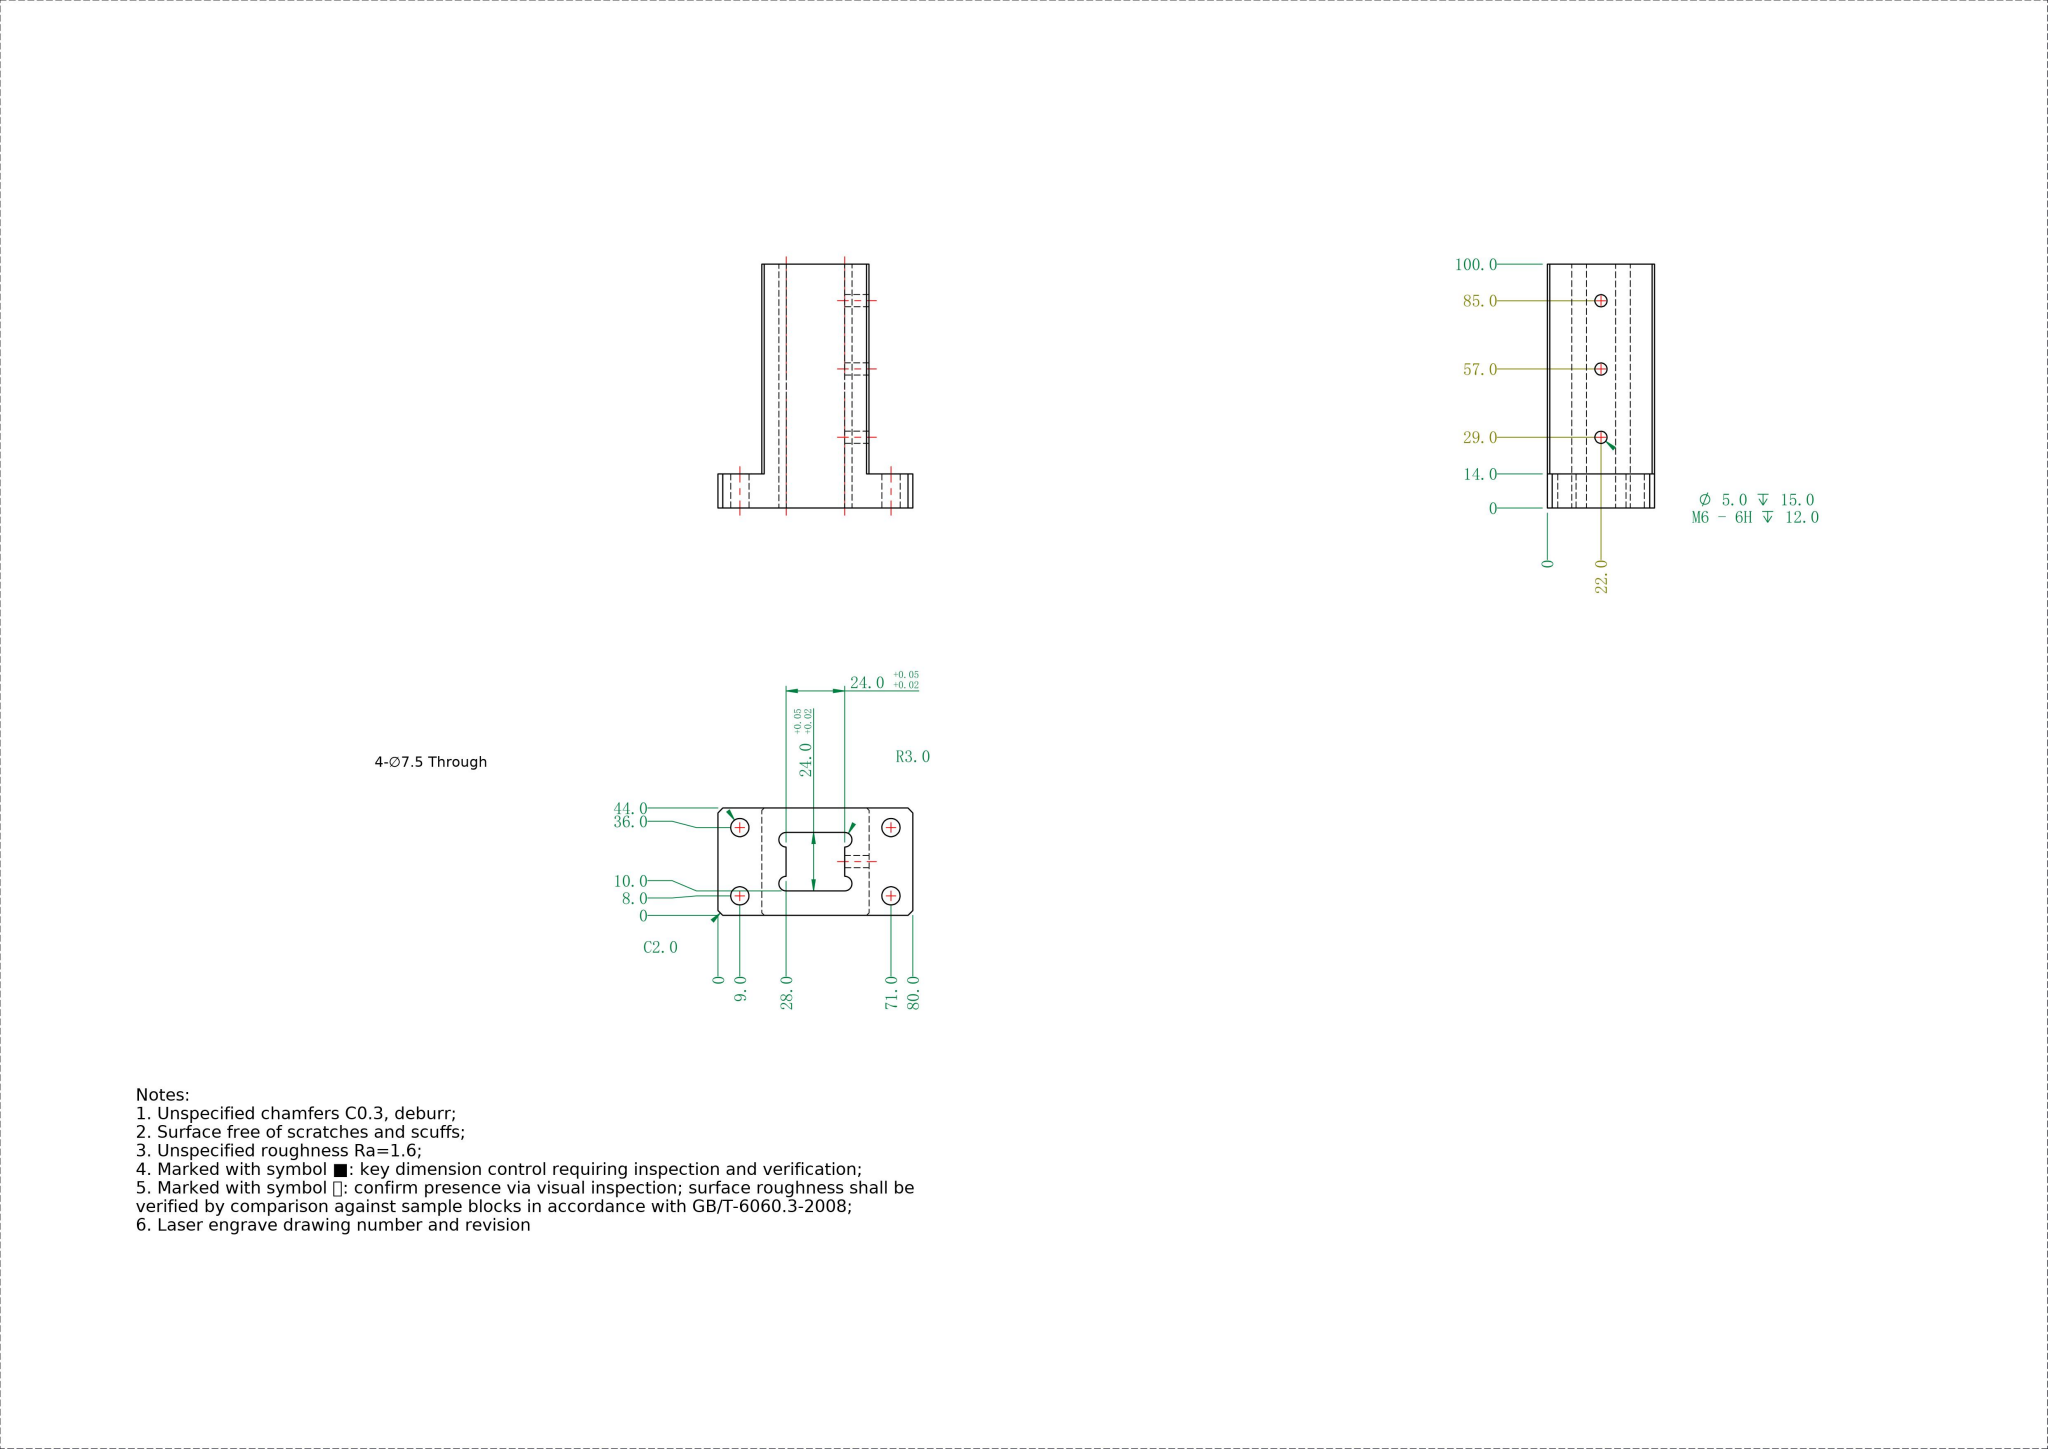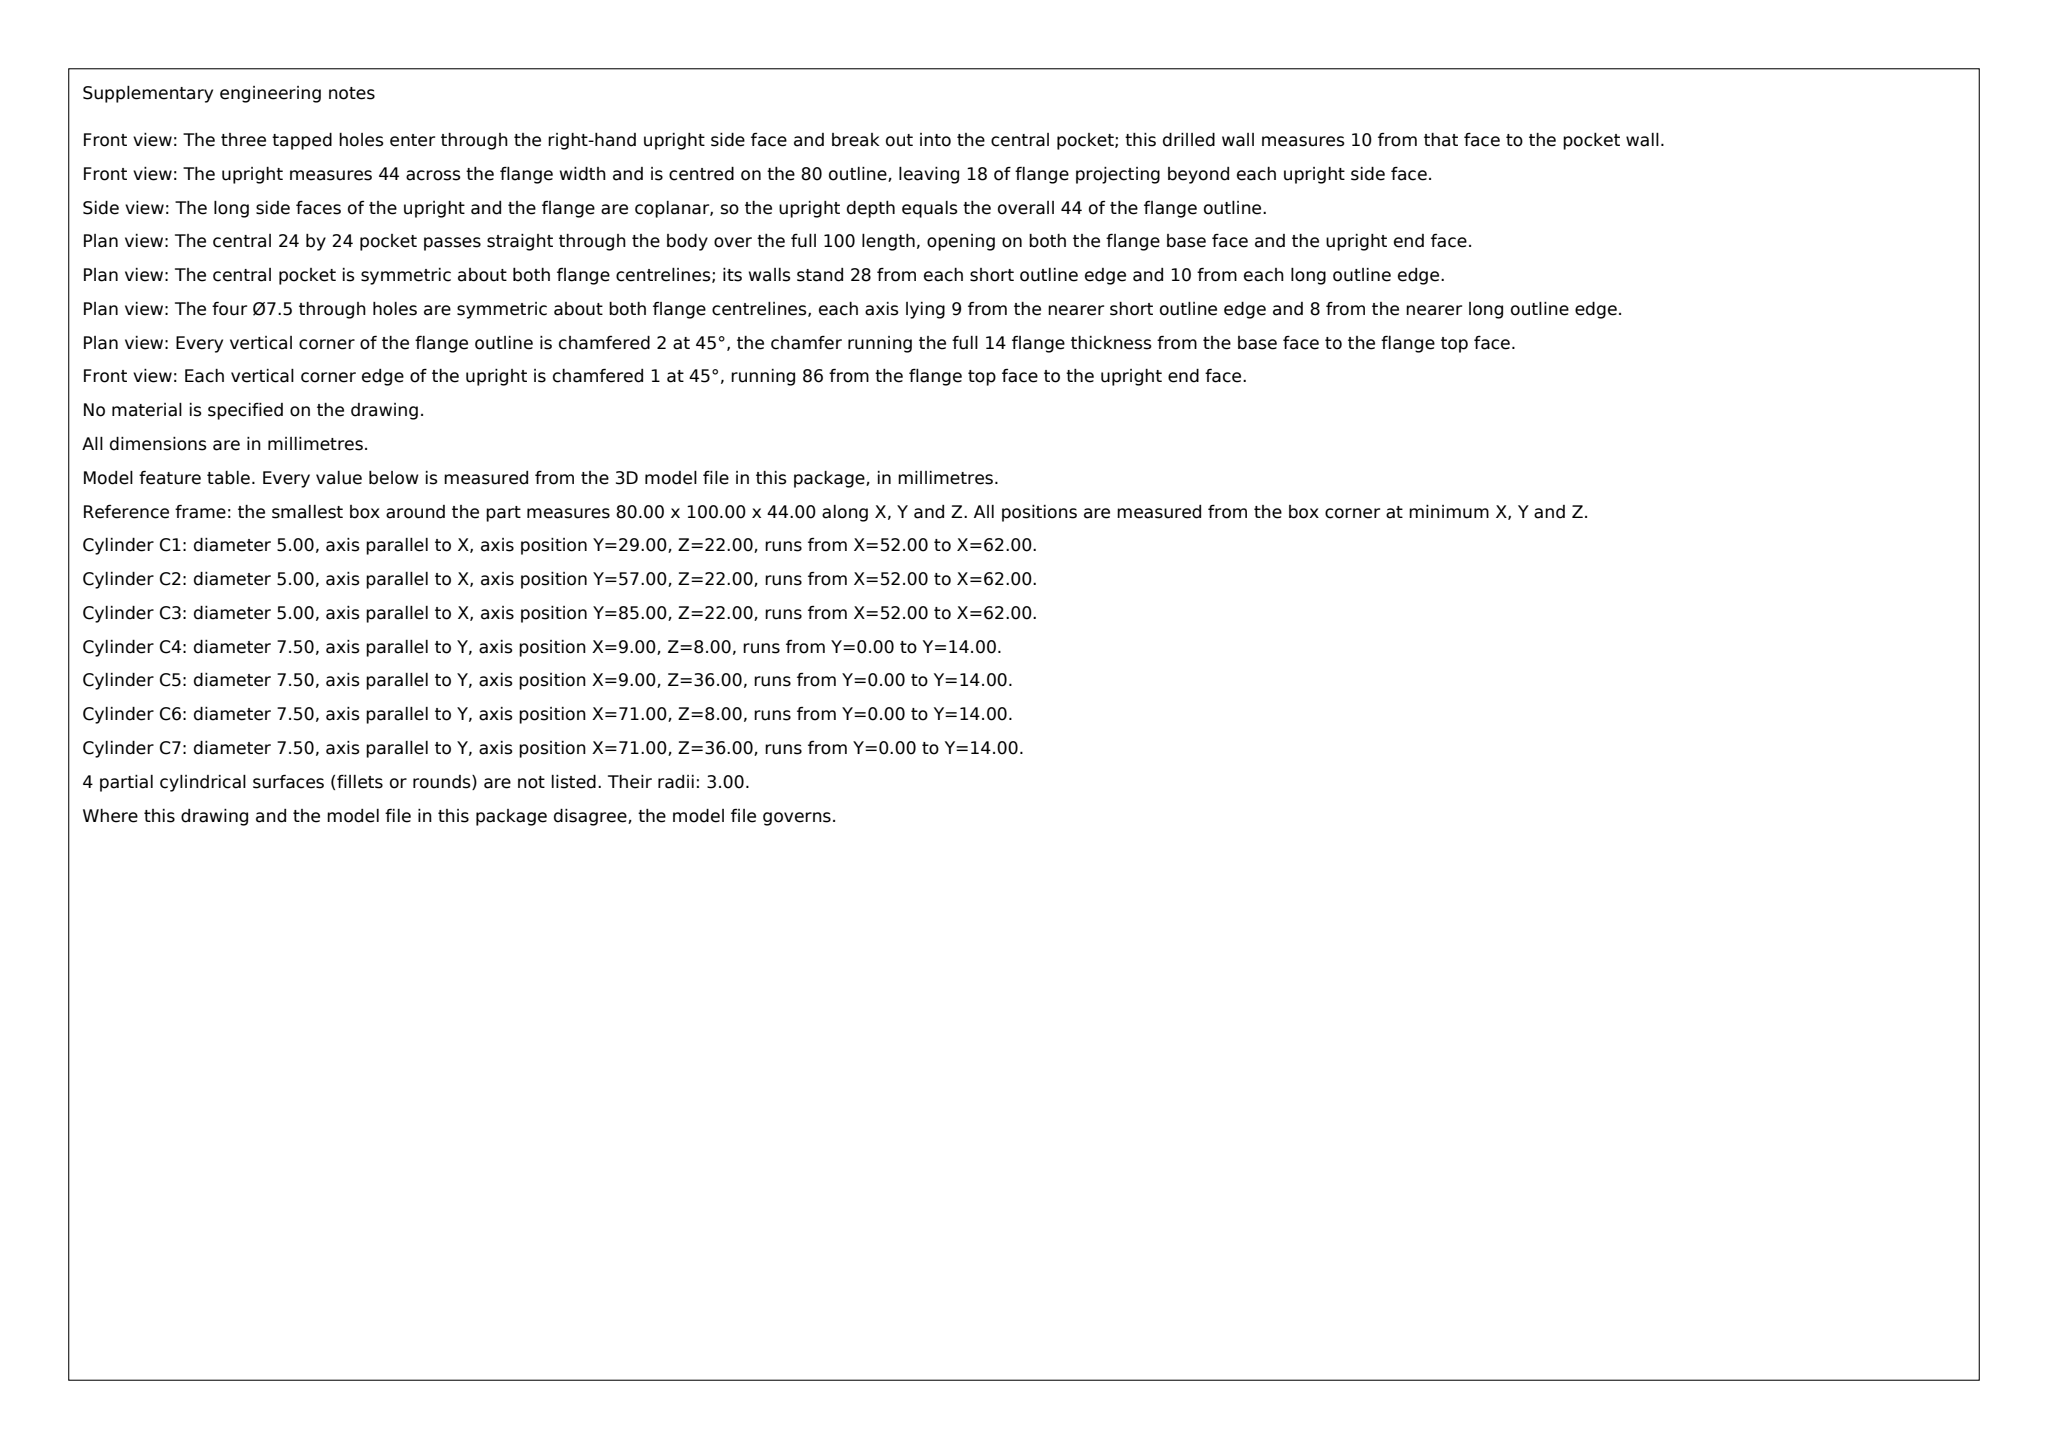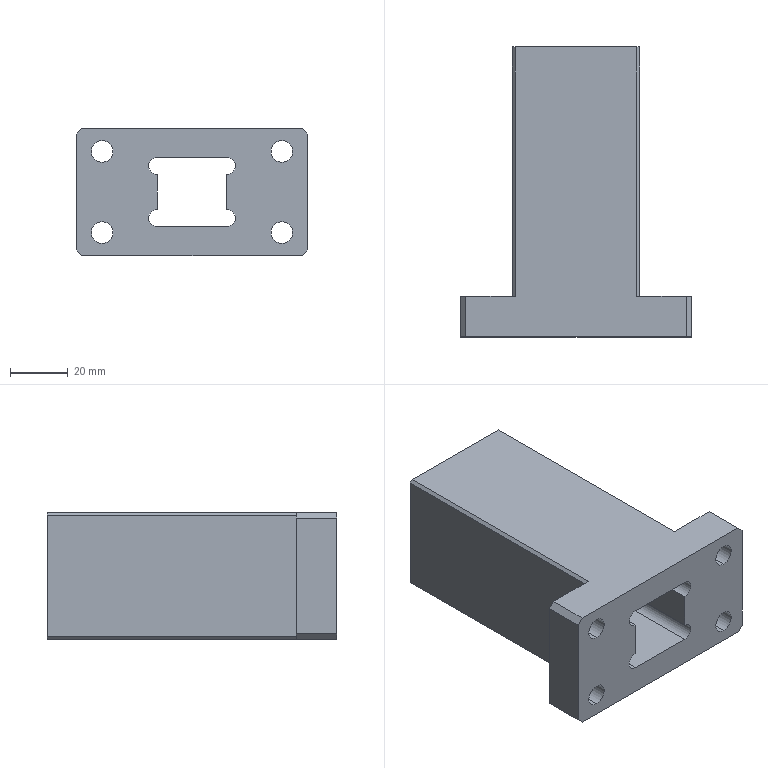Part | SolidWorks | mm | 1 solid | 40 faces | box 80 x 100 x 44 mm | volume 149174 mm3 | plane 22 | cylinder 18 | commonest cylinder face diameters 7.5 x8 5 x6 6 x4
Drawing notes:
STOCK 80.0 x 100.0 x 44.0 | from the solid: bbox_xyz 80.0, 100.0, 44.0
UPRIGHT 44.0 WIDE, WALL THK 10.0 EA SIDE OF 24.0 SLOT | from the solid: x planes 18.0/28.0 and 52.0/62.0 = 10.0 wall; upright 18-62 = 44.0; slot 28-52 = 24.0
SLOT 24.0 x 24.0 THRU 100.0, R3.0 CNRS | from the solid: slot x 28-52, z 10-34, full y length 100.0; R3.0 on sheet 1
4X Ø6.0 CNR RELIEF THRU 100.0 AT SLOT CNRS | from the solid: cylinders dia 6.0 axis y, length 100.0, at (28/52, 13/31)
6X Ø5.0 DP 15.0, M6-6H DP 12.0: 3 PER WALL, BOTH WALLS | from the solid: dia 5.0 axis x at y=29/57/85, z=22, count 2 each = 6 total
4X Ø6.0 THRU: X=28.0 & 52.0, Z=13.0 & 31.0 (PLAN VIEW 0 DATUMS) | from the solid: cyl dia 6.0 axis y at (x,z)=(28,13),(28,31),(52,13),(52,31), len 100 thru; slot walls x=28/52, slot faces z=10/34
4X C2.0 AT PLATE CORNERS, 80.0 X 44.0 OUTLINE (PLAN VIEW) | from the solid: bbox 80.0 x 44.0 in X-Z; outer planes x=0/80, z=0/44; corner cuts not axis-aligned
4X C1.0 ON VERT EDGES OF 24.0 SQ COLUMN, Y 14.0 TO 100.0 | from the solid: column planes x=28/52 and z=10/34 (24.0 sq) between y=14 flange face and y=100 top
build123d program:
from build123d import *

# Parameters (mm, degrees)
SKETCH1_W             = 80
SKETCH1_H             = 44
BOSS_EXTRUDE1_DEPTH   = 100
SKETCH2_W             = 24
SKETCH2_H             = 24
CUT_EXTRUDE1_DEPTH    = 110.927
SKETCH6_W             = 18
SKETCH6_H             = 44
CUT_EXTRUDE4_DEPTH    = 86
SKETCH7_R             = 3.75
CUT_EXTRUDE5_DEPTH    = 98.365
CHAMFER1_SIZE         = 2
CHAMFER2_SIZE         = 1
SKETCH8_R             = 3
CUT_EXTRUDE6_DEPTH    = 110.927
M6_TAPPED_HOLE1_D     = 5
M6_TAPPED_HOLE1_DEPTH = 15
M6_TAPPED_HOLE1_TIP   = 1.502


with BuildPart() as part:
    # Sketch1 → Boss-Extrude1 (new body)
    with BuildSketch(Plane(origin=(0, 0, 0), x_dir=(1, 0, 0), z_dir=(0, 1, 0))):
        Rectangle(SKETCH1_W, SKETCH1_H)
    extrude(amount=BOSS_EXTRUDE1_DEPTH)

    # Sketch2 → Cut-Extrude1 (cut, through all)
    with BuildSketch(Plane(origin=(0, 100, 0), x_dir=(1, 0, 0), z_dir=(0, 1, 0))):
        Rectangle(SKETCH2_W, SKETCH2_H)
    extrude(amount=-CUT_EXTRUDE1_DEPTH, mode=Mode.SUBTRACT)

    # Sketch6 → Cut-Extrude4 (cut)
    with BuildSketch(Plane(origin=(0, 100, 0), x_dir=(1, 0, 0), z_dir=(0, 1, 0))):
        with Locations((-31, 0)):
            Rectangle(SKETCH6_W, SKETCH6_H)
        with Locations((31, 0)):
            Rectangle(SKETCH6_W, SKETCH6_H)
    extrude(amount=-CUT_EXTRUDE4_DEPTH, mode=Mode.SUBTRACT)

    # Sketch7 → Cut-Extrude5 (cut, through all)
    with BuildSketch(Plane(origin=(0, 14, 0), x_dir=(1, 0, 0), z_dir=(0, 1, 0))):
        with Locations(Location((-31, -14, 0), (0, 0, 270))):
            Circle(SKETCH7_R)
        with Locations(Location((-31, 14, 0), (0, 0, 270))):
            Circle(SKETCH7_R)
        with Locations(Location((31, -14, 0), (0, 0, 270))):
            Circle(SKETCH7_R)
        with Locations(Location((31, 14, 0), (0, 0, 270))):
            Circle(SKETCH7_R)
    extrude(amount=-CUT_EXTRUDE5_DEPTH, mode=Mode.SUBTRACT)

    # Chamfer1
    chamfer1_edges = [part.edges().sort_by_distance(p)[0] for p in [
        (40, 7, 22),
        (-40, 7, 22),
        (-40, 7, -22),
        (40, 7, -22),
    ]]
    chamfer(chamfer1_edges, length=CHAMFER1_SIZE)

    # Chamfer2
    chamfer2_edges = [part.edges().sort_by_distance(p)[0] for p in [
        (-22, 57, -22),
        (-22, 57, 22),
        (22, 57, 22),
        (22, 57, -22),
    ]]
    chamfer(chamfer2_edges, length=CHAMFER2_SIZE)

    # Sketch8 → Cut-Extrude6 (cut, through all)
    with BuildSketch(Plane(origin=(0, 100, 0), x_dir=(1, 0, 0), z_dir=(0, 1, 0))):
        with Locations((-12, 9)):
            Circle(SKETCH8_R)
        with Locations((-12, -9)):
            Circle(SKETCH8_R)
        with Locations((12, -9)):
            Circle(SKETCH8_R)
        with Locations((12, 9)):
            Circle(SKETCH8_R)
    extrude(amount=-CUT_EXTRUDE6_DEPTH, mode=Mode.SUBTRACT)

    # M6 Tapped Hole1
    with Locations(Plane(origin=(22, 0, 0), x_dir=(0, 0, -1), z_dir=(1, 0, 0))):
        with Locations((0, 85), (0, 57), (0, 29)):
            Hole(M6_TAPPED_HOLE1_D / 2, depth=M6_TAPPED_HOLE1_DEPTH)
            with Locations((0, 0, -(M6_TAPPED_HOLE1_DEPTH + M6_TAPPED_HOLE1_TIP / 2))):  # 118° drill point
                Cone(0, M6_TAPPED_HOLE1_D / 2, M6_TAPPED_HOLE1_TIP, mode=Mode.SUBTRACT)


solid = part.part